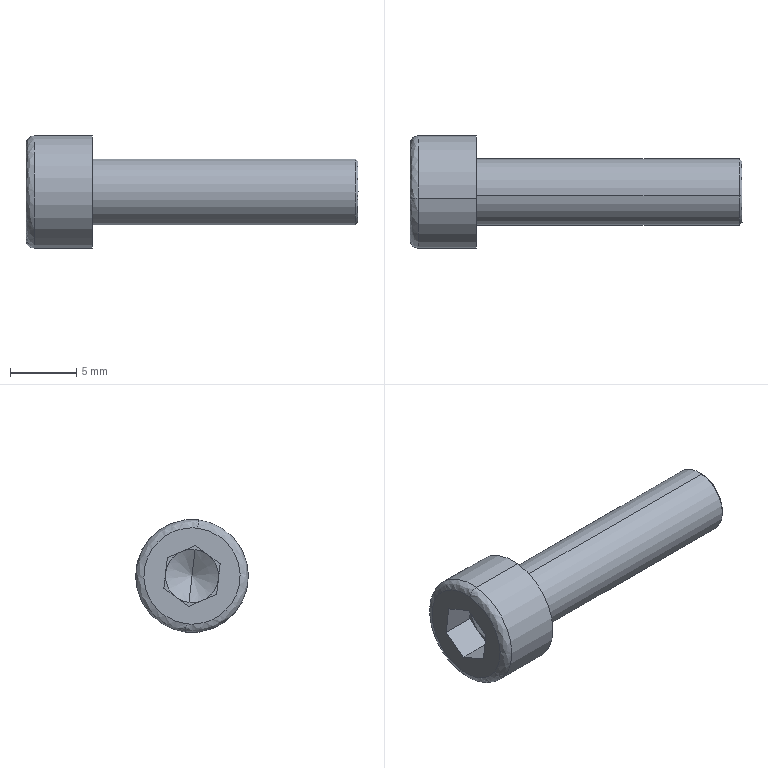Component | SolidWorks | V1ZHXTRR60SecondarySB1-1_v1ZHXTHexagon socket head cap screws GB_GB_FASTENER_SCREWS_HSHCS M5X20-N_1SB1-1 | 1 solid | 25 faces | box 25 x 8.5 x 8.5 mm | volume 634 mm3 | plane 15 | cylinder 4 | cone 4 | spline 2 | commonest cylinder face diameters 5 x2 8.5 x2
STEP:
#1=CARTESIAN_POINT('',(3.529,-7.033,21.044));
#2=VERTEX_POINT('',#1);
#3=CARTESIAN_POINT('',(3.529,-7.072,21.376));
#4=VERTEX_POINT('',#3);
#5=CARTESIAN_POINT('',(3.529,-7.052,21.21));
#6=DIRECTION('',(1.,0.,-0.));
#7=DIRECTION('',(-0.,0.1167,-0.9932));
#8=AXIS2_PLACEMENT_3D('',#5,#6,#7);
#9=CIRCLE('',#8,0.1673);
#10=EDGE_CURVE('',#2,#4,#9,.T.);
#11=ORIENTED_EDGE('',*,*,#10,.F.);
#12=CARTESIAN_POINT('',(3.505,-7.036,21.068));
#13=VERTEX_POINT('',#12);
#14=CARTESIAN_POINT('',(3.529,-7.036,21.068));
#15=DIRECTION('',(-0.,0.9932,0.1167));
#16=DIRECTION('',(-0.,0.1167,-0.9932));
#17=AXIS2_PLACEMENT_3D('',#14,#15,#16);
#18=CIRCLE('',#17,0.02461);
#19=EDGE_CURVE('',#2,#13,#18,.T.);
#20=ORIENTED_EDGE('',*,*,#19,.T.);
#21=CARTESIAN_POINT('',(3.505,-7.069,21.352));
#22=VERTEX_POINT('',#21);
#23=CARTESIAN_POINT('',(3.505,-7.036,21.068));
#24=CARTESIAN_POINT('',(3.505,-6.752,21.102));
#25=CARTESIAN_POINT('',(3.505,-6.786,21.385));
#26=CARTESIAN_POINT('',(3.505,-7.069,21.352));
#27=(BOUNDED_CURVE()B_SPLINE_CURVE(3,(#23,#24,#25,#26),.UNSPECIFIED.,.F.,.F.)B_SPLINE_CURVE_WITH_KNOTS((4,4),(0.,1.),.UNSPECIFIED.)CURVE()GEOMETRIC_REPRESENTATION_ITEM()RATIONAL_B_SPLINE_CURVE((1.,0.3333,0.3333,1.))REPRESENTATION_ITEM(''));
#28=EDGE_CURVE('',#13,#22,#27,.T.);
#29=ORIENTED_EDGE('',*,*,#28,.T.);
#30=CARTESIAN_POINT('',(3.529,-7.069,21.352));
#31=DIRECTION('',(0.,-0.9932,-0.1167));
#32=DIRECTION('',(0.,-0.1167,0.9932));
#33=AXIS2_PLACEMENT_3D('',#30,#31,#32);
#34=CIRCLE('',#33,0.02461);
#35=EDGE_CURVE('',#4,#22,#34,.T.);
#36=ORIENTED_EDGE('',*,*,#35,.F.);
#37=EDGE_LOOP('',(#11,#20,#29,#36));
#38=FACE_OUTER_BOUND('',#37,.T.);
#39=CARTESIAN_POINT('',(3.529,-7.033,21.044));
#40=CARTESIAN_POINT('',(3.529,-6.701,21.083));
#41=CARTESIAN_POINT('',(3.529,-6.74,21.415));
#42=CARTESIAN_POINT('',(3.529,-7.072,21.376));
#43=CARTESIAN_POINT('',(3.515,-7.033,21.044));
#44=CARTESIAN_POINT('',(3.515,-6.701,21.083));
#45=CARTESIAN_POINT('',(3.515,-6.74,21.415));
#46=CARTESIAN_POINT('',(3.515,-7.072,21.376));
#47=CARTESIAN_POINT('',(3.505,-7.034,21.054));
#48=CARTESIAN_POINT('',(3.505,-6.722,21.091));
#49=CARTESIAN_POINT('',(3.505,-6.759,21.403));
#50=CARTESIAN_POINT('',(3.505,-7.071,21.366));
#51=CARTESIAN_POINT('',(3.505,-7.036,21.068));
#52=CARTESIAN_POINT('',(3.505,-6.752,21.102));
#53=CARTESIAN_POINT('',(3.505,-6.786,21.385));
#54=CARTESIAN_POINT('',(3.505,-7.069,21.352));
#55=(BOUNDED_SURFACE()B_SPLINE_SURFACE(3,3,((#39,#40,#41,#42),(#43,#44,#45,#46),(#47,#48,#49,#50),(#51,#52,#53,#54)),.UNSPECIFIED.,.F.,.F.,.F.)B_SPLINE_SURFACE_WITH_KNOTS((4,4),(4,4),(0.,1.),(0.,1.),.UNSPECIFIED.)GEOMETRIC_REPRESENTATION_ITEM()RATIONAL_B_SPLINE_SURFACE(((1.,0.3333,0.3333,1.),(0.8047,0.2682,0.2682,0.8047),(0.8047,0.2682,0.2682,0.8047),(1.,0.3333,0.3333,1.)))REPRESENTATION_ITEM('')SURFACE());
#56=ADVANCED_FACE('',(#38),#55,.T.);
#57=CARTESIAN_POINT('',(4.481,-7.041,21.112));
#58=VERTEX_POINT('',#57);
#59=CARTESIAN_POINT('',(4.481,-7.064,21.308));
#60=VERTEX_POINT('',#59);
#61=CARTESIAN_POINT('',(4.481,-7.052,21.21));
#62=DIRECTION('',(-1.,-0.,0.));
#63=DIRECTION('',(-0.,0.1167,-0.9932));
#64=AXIS2_PLACEMENT_3D('',#61,#62,#63);
#65=CIRCLE('',#64,0.09843);
#66=EDGE_CURVE('',#58,#60,#65,.T.);
#67=ORIENTED_EDGE('',*,*,#66,.T.);
#68=CARTESIAN_POINT('',(3.702,-7.064,21.308));
#69=VERTEX_POINT('',#68);
#70=CARTESIAN_POINT('',(4.489,-7.064,21.308));
#71=DIRECTION('',(-1.,-0.,0.));
#72=VECTOR('',#71,39.37);
#73=LINE('',#70,#72);
#74=EDGE_CURVE('',#60,#69,#73,.T.);
#75=ORIENTED_EDGE('',*,*,#74,.T.);
#76=CARTESIAN_POINT('',(3.702,-7.041,21.112));
#77=VERTEX_POINT('',#76);
#78=CARTESIAN_POINT('',(3.702,-7.052,21.21));
#79=DIRECTION('',(1.,0.,-0.));
#80=DIRECTION('',(-0.,0.1167,-0.9932));
#81=AXIS2_PLACEMENT_3D('',#78,#79,#80);
#82=CIRCLE('',#81,0.09843);
#83=EDGE_CURVE('',#69,#77,#82,.T.);
#84=ORIENTED_EDGE('',*,*,#83,.T.);
#85=CARTESIAN_POINT('',(4.489,-7.041,21.112));
#86=DIRECTION('',(-1.,-0.,0.));
#87=VECTOR('',#86,39.37);
#88=LINE('',#85,#87);
#89=EDGE_CURVE('',#58,#77,#88,.T.);
#90=ORIENTED_EDGE('',*,*,#89,.F.);
#91=EDGE_LOOP('',(#67,#75,#84,#90));
#92=FACE_OUTER_BOUND('',#91,.T.);
#93=CARTESIAN_POINT('',(4.489,-7.052,21.21));
#94=DIRECTION('',(-1.,-0.,0.));
#95=DIRECTION('',(-0.,0.1167,-0.9932));
#96=AXIS2_PLACEMENT_3D('',#93,#94,#95);
#97=CYLINDRICAL_SURFACE('',#96,0.09843);
#98=ADVANCED_FACE('',(#92),#97,.T.);
#99=CARTESIAN_POINT('',(4.489,-7.042,21.12));
#100=VERTEX_POINT('',#99);
#101=CARTESIAN_POINT('',(4.489,-7.063,21.3));
#102=VERTEX_POINT('',#101);
#103=CARTESIAN_POINT('',(4.489,-7.052,21.21));
#104=DIRECTION('',(-1.,-0.,0.));
#105=DIRECTION('',(-0.,0.1167,-0.9932));
#106=AXIS2_PLACEMENT_3D('',#103,#104,#105);
#107=CIRCLE('',#106,0.09055);
#108=EDGE_CURVE('',#100,#102,#107,.T.);
#109=ORIENTED_EDGE('',*,*,#108,.T.);
#110=CARTESIAN_POINT('',(4.481,-7.064,21.308));
#111=DIRECTION('',(-0.7071,-0.0825,0.7023));
#112=VECTOR('',#111,39.37);
#113=LINE('',#110,#112);
#114=EDGE_CURVE('',#102,#60,#113,.T.);
#115=ORIENTED_EDGE('',*,*,#114,.T.);
#116=ORIENTED_EDGE('',*,*,#66,.F.);
#117=CARTESIAN_POINT('',(4.481,-7.041,21.112));
#118=DIRECTION('',(-0.7071,0.0825,-0.7023));
#119=VECTOR('',#118,39.37);
#120=LINE('',#117,#119);
#121=EDGE_CURVE('',#100,#58,#120,.T.);
#122=ORIENTED_EDGE('',*,*,#121,.F.);
#123=EDGE_LOOP('',(#109,#115,#116,#122));
#124=FACE_OUTER_BOUND('',#123,.T.);
#125=CARTESIAN_POINT('',(4.481,-7.052,21.21));
#126=DIRECTION('',(-1.,-0.,0.));
#127=DIRECTION('',(-0.,0.1167,-0.9932));
#128=AXIS2_PLACEMENT_3D('',#125,#126,#127);
#129=CONICAL_SURFACE('',#128,0.09843,0.7854);
#130=ADVANCED_FACE('',(#124),#129,.T.);
#131=CARTESIAN_POINT('',(3.702,-7.072,21.376));
#132=VERTEX_POINT('',#131);
#133=CARTESIAN_POINT('',(3.702,-7.033,21.044));
#134=VERTEX_POINT('',#133);
#135=CARTESIAN_POINT('',(3.702,-7.052,21.21));
#136=DIRECTION('',(1.,0.,-0.));
#137=DIRECTION('',(-0.,0.1167,-0.9932));
#138=AXIS2_PLACEMENT_3D('',#135,#136,#137);
#139=CIRCLE('',#138,0.1673);
#140=EDGE_CURVE('',#132,#134,#139,.T.);
#141=ORIENTED_EDGE('',*,*,#140,.F.);
#142=CARTESIAN_POINT('',(3.702,-7.072,21.376));
#143=DIRECTION('',(-1.,-0.,0.));
#144=VECTOR('',#143,39.37);
#145=LINE('',#142,#144);
#146=EDGE_CURVE('',#132,#4,#145,.T.);
#147=ORIENTED_EDGE('',*,*,#146,.T.);
#148=CARTESIAN_POINT('',(3.529,-7.052,21.21));
#149=DIRECTION('',(1.,0.,-0.));
#150=DIRECTION('',(-0.,0.1167,-0.9932));
#151=AXIS2_PLACEMENT_3D('',#148,#149,#150);
#152=CIRCLE('',#151,0.1673);
#153=EDGE_CURVE('',#4,#2,#152,.T.);
#154=ORIENTED_EDGE('',*,*,#153,.T.);
#155=CARTESIAN_POINT('',(3.702,-7.033,21.044));
#156=DIRECTION('',(-1.,-0.,0.));
#157=VECTOR('',#156,39.37);
#158=LINE('',#155,#157);
#159=EDGE_CURVE('',#134,#2,#158,.T.);
#160=ORIENTED_EDGE('',*,*,#159,.F.);
#161=EDGE_LOOP('',(#141,#147,#154,#160));
#162=FACE_OUTER_BOUND('',#161,.T.);
#163=CARTESIAN_POINT('',(3.702,-7.052,21.21));
#164=DIRECTION('',(-1.,-0.,0.));
#165=DIRECTION('',(-0.,0.1167,-0.9932));
#166=AXIS2_PLACEMENT_3D('',#163,#164,#165);
#167=CYLINDRICAL_SURFACE('',#166,0.1673);
#168=ADVANCED_FACE('',(#162),#167,.T.);
#169=CARTESIAN_POINT('',(3.649,-7.052,21.21));
#170=VERTEX_POINT('',#169);
#171=CARTESIAN_POINT('',(3.603,-7.043,21.132));
#172=VERTEX_POINT('',#171);
#173=CARTESIAN_POINT('',(3.603,-7.043,21.132));
#174=DIRECTION('',(-0.5,0.101,-0.8601));
#175=VECTOR('',#174,39.37);
#176=LINE('',#173,#175);
#177=EDGE_CURVE('',#170,#172,#176,.T.);
#178=ORIENTED_EDGE('',*,*,#177,.F.);
#179=CARTESIAN_POINT('',(3.603,-7.062,21.288));
#180=VERTEX_POINT('',#179);
#181=CARTESIAN_POINT('',(3.603,-7.062,21.288));
#182=DIRECTION('',(-0.5,-0.101,0.8601));
#183=VECTOR('',#182,39.37);
#184=LINE('',#181,#183);
#185=EDGE_CURVE('',#170,#180,#184,.T.);
#186=ORIENTED_EDGE('',*,*,#185,.T.);
#187=CARTESIAN_POINT('',(3.603,-7.021,21.283));
#188=VERTEX_POINT('',#187);
#189=CARTESIAN_POINT('',(3.603,-7.052,21.21));
#190=DIRECTION('',(1.,0.,-0.));
#191=DIRECTION('',(-0.,0.1167,-0.9932));
#192=AXIS2_PLACEMENT_3D('',#189,#190,#191);
#193=CIRCLE('',#192,0.07874);
#194=EDGE_CURVE('',#188,#180,#193,.T.);
#195=ORIENTED_EDGE('',*,*,#194,.F.);
#196=CARTESIAN_POINT('',(3.603,-6.974,21.219));
#197=VERTEX_POINT('',#196);
#198=CARTESIAN_POINT('',(3.603,-7.052,21.21));
#199=DIRECTION('',(1.,0.,-0.));
#200=DIRECTION('',(-0.,0.1167,-0.9932));
#201=AXIS2_PLACEMENT_3D('',#198,#199,#200);
#202=CIRCLE('',#201,0.07874);
#203=EDGE_CURVE('',#197,#188,#202,.T.);
#204=ORIENTED_EDGE('',*,*,#203,.F.);
#205=CARTESIAN_POINT('',(3.603,-7.005,21.147));
#206=VERTEX_POINT('',#205);
#207=CARTESIAN_POINT('',(3.603,-7.052,21.21));
#208=DIRECTION('',(-1.,-0.,0.));
#209=DIRECTION('',(-0.,0.1167,-0.9932));
#210=AXIS2_PLACEMENT_3D('',#207,#208,#209);
#211=CIRCLE('',#210,0.07874);
#212=EDGE_CURVE('',#197,#206,#211,.T.);
#213=ORIENTED_EDGE('',*,*,#212,.T.);
#214=CARTESIAN_POINT('',(3.603,-7.052,21.21));
#215=DIRECTION('',(1.,0.,-0.));
#216=DIRECTION('',(-0.,0.1167,-0.9932));
#217=AXIS2_PLACEMENT_3D('',#214,#215,#216);
#218=CIRCLE('',#217,0.07874);
#219=EDGE_CURVE('',#172,#206,#218,.T.);
#220=ORIENTED_EDGE('',*,*,#219,.F.);
#221=EDGE_LOOP('',(#178,#186,#195,#204,#213,#220));
#222=FACE_OUTER_BOUND('',#221,.T.);
#223=CARTESIAN_POINT('',(3.603,-7.052,21.21));
#224=DIRECTION('',(-1.,-0.,0.));
#225=DIRECTION('',(-0.,0.1167,-0.9932));
#226=AXIS2_PLACEMENT_3D('',#223,#224,#225);
#227=CONICAL_SURFACE('',#226,0.07874,1.047);
#228=ADVANCED_FACE('',(#222),#227,.F.);
#229=ORIENTED_EDGE('',*,*,#74,.F.);
#230=CARTESIAN_POINT('',(4.481,-7.052,21.21));
#231=DIRECTION('',(-1.,-0.,0.));
#232=DIRECTION('',(-0.,0.1167,-0.9932));
#233=AXIS2_PLACEMENT_3D('',#230,#231,#232);
#234=CIRCLE('',#233,0.09843);
#235=EDGE_CURVE('',#60,#58,#234,.T.);
#236=ORIENTED_EDGE('',*,*,#235,.T.);
#237=ORIENTED_EDGE('',*,*,#89,.T.);
#238=CARTESIAN_POINT('',(3.702,-7.052,21.21));
#239=DIRECTION('',(1.,0.,-0.));
#240=DIRECTION('',(-0.,0.1167,-0.9932));
#241=AXIS2_PLACEMENT_3D('',#238,#239,#240);
#242=CIRCLE('',#241,0.09843);
#243=EDGE_CURVE('',#77,#69,#242,.T.);
#244=ORIENTED_EDGE('',*,*,#243,.T.);
#245=EDGE_LOOP('',(#229,#236,#237,#244));
#246=FACE_OUTER_BOUND('',#245,.T.);
#247=CARTESIAN_POINT('',(4.489,-7.052,21.21));
#248=DIRECTION('',(-1.,-0.,0.));
#249=DIRECTION('',(-0.,0.1167,-0.9932));
#250=AXIS2_PLACEMENT_3D('',#247,#248,#249);
#251=CYLINDRICAL_SURFACE('',#250,0.09843);
#252=ADVANCED_FACE('',(#246),#251,.T.);
#253=ORIENTED_EDGE('',*,*,#243,.F.);
#254=ORIENTED_EDGE('',*,*,#83,.F.);
#255=EDGE_LOOP('',(#253,#254));
#256=FACE_BOUND('',#255,.T.);
#257=CARTESIAN_POINT('',(3.702,-7.052,21.21));
#258=DIRECTION('',(1.,0.,-0.));
#259=DIRECTION('',(-0.,0.1167,-0.9932));
#260=AXIS2_PLACEMENT_3D('',#257,#258,#259);
#261=CIRCLE('',#260,0.1673);
#262=EDGE_CURVE('',#134,#132,#261,.T.);
#263=ORIENTED_EDGE('',*,*,#262,.T.);
#264=ORIENTED_EDGE('',*,*,#140,.T.);
#265=EDGE_LOOP('',(#263,#264));
#266=FACE_OUTER_BOUND('',#265,.T.);
#267=CARTESIAN_POINT('',(3.702,-7.052,21.21));
#268=DIRECTION('',(1.,0.,-0.));
#269=DIRECTION('',(0.,-0.1167,0.9932));
#270=AXIS2_PLACEMENT_3D('',#267,#268,#269);
#271=PLANE('',#270);
#272=ADVANCED_FACE('',(#256,#266),#271,.T.);
#273=ORIENTED_EDGE('',*,*,#114,.F.);
#274=CARTESIAN_POINT('',(4.489,-7.052,21.21));
#275=DIRECTION('',(-1.,-0.,0.));
#276=DIRECTION('',(-0.,0.1167,-0.9932));
#277=AXIS2_PLACEMENT_3D('',#274,#275,#276);
#278=CIRCLE('',#277,0.09055);
#279=EDGE_CURVE('',#102,#100,#278,.T.);
#280=ORIENTED_EDGE('',*,*,#279,.T.);
#281=ORIENTED_EDGE('',*,*,#121,.T.);
#282=ORIENTED_EDGE('',*,*,#235,.F.);
#283=EDGE_LOOP('',(#273,#280,#281,#282));
#284=FACE_OUTER_BOUND('',#283,.T.);
#285=CARTESIAN_POINT('',(4.481,-7.052,21.21));
#286=DIRECTION('',(-1.,-0.,0.));
#287=DIRECTION('',(-0.,0.1167,-0.9932));
#288=AXIS2_PLACEMENT_3D('',#285,#286,#287);
#289=CONICAL_SURFACE('',#288,0.09843,0.7854);
#290=ADVANCED_FACE('',(#284),#289,.T.);
#291=ORIENTED_EDGE('',*,*,#146,.F.);
#292=ORIENTED_EDGE('',*,*,#262,.F.);
#293=ORIENTED_EDGE('',*,*,#159,.T.);
#294=ORIENTED_EDGE('',*,*,#10,.T.);
#295=EDGE_LOOP('',(#291,#292,#293,#294));
#296=FACE_OUTER_BOUND('',#295,.T.);
#297=CARTESIAN_POINT('',(3.702,-7.052,21.21));
#298=DIRECTION('',(-1.,-0.,0.));
#299=DIRECTION('',(-0.,0.1167,-0.9932));
#300=AXIS2_PLACEMENT_3D('',#297,#298,#299);
#301=CYLINDRICAL_SURFACE('',#300,0.1673);
#302=ADVANCED_FACE('',(#296),#301,.T.);
#303=ORIENTED_EDGE('',*,*,#108,.F.);
#304=ORIENTED_EDGE('',*,*,#279,.F.);
#305=EDGE_LOOP('',(#303,#304));
#306=FACE_OUTER_BOUND('',#305,.T.);
#307=CARTESIAN_POINT('',(4.489,-7.052,21.21));
#308=DIRECTION('',(1.,0.,-0.));
#309=DIRECTION('',(0.,-0.1167,0.9932));
#310=AXIS2_PLACEMENT_3D('',#307,#308,#309);
#311=PLANE('',#310);
#312=ADVANCED_FACE('',(#306),#311,.T.);
#313=ORIENTED_EDGE('',*,*,#19,.F.);
#314=ORIENTED_EDGE('',*,*,#153,.F.);
#315=ORIENTED_EDGE('',*,*,#35,.T.);
#316=CARTESIAN_POINT('',(3.505,-7.069,21.352));
#317=CARTESIAN_POINT('',(3.505,-7.353,21.319));
#318=CARTESIAN_POINT('',(3.505,-7.319,21.035));
#319=CARTESIAN_POINT('',(3.505,-7.036,21.068));
#320=(BOUNDED_CURVE()B_SPLINE_CURVE(3,(#316,#317,#318,#319),.UNSPECIFIED.,.F.,.F.)B_SPLINE_CURVE_WITH_KNOTS((4,4),(0.,1.),.UNSPECIFIED.)CURVE()GEOMETRIC_REPRESENTATION_ITEM()RATIONAL_B_SPLINE_CURVE((1.,0.3333,0.3333,1.))REPRESENTATION_ITEM(''));
#321=EDGE_CURVE('',#22,#13,#320,.T.);
#322=ORIENTED_EDGE('',*,*,#321,.T.);
#323=EDGE_LOOP('',(#313,#314,#315,#322));
#324=FACE_OUTER_BOUND('',#323,.T.);
#325=CARTESIAN_POINT('',(3.529,-7.072,21.376));
#326=CARTESIAN_POINT('',(3.529,-7.404,21.337));
#327=CARTESIAN_POINT('',(3.529,-7.365,21.005));
#328=CARTESIAN_POINT('',(3.529,-7.033,21.044));
#329=CARTESIAN_POINT('',(3.515,-7.072,21.376));
#330=CARTESIAN_POINT('',(3.515,-7.404,21.337));
#331=CARTESIAN_POINT('',(3.515,-7.365,21.005));
#332=CARTESIAN_POINT('',(3.515,-7.033,21.044));
#333=CARTESIAN_POINT('',(3.505,-7.071,21.366));
#334=CARTESIAN_POINT('',(3.505,-7.383,21.33));
#335=CARTESIAN_POINT('',(3.505,-7.346,21.017));
#336=CARTESIAN_POINT('',(3.505,-7.034,21.054));
#337=CARTESIAN_POINT('',(3.505,-7.069,21.352));
#338=CARTESIAN_POINT('',(3.505,-7.353,21.319));
#339=CARTESIAN_POINT('',(3.505,-7.319,21.035));
#340=CARTESIAN_POINT('',(3.505,-7.036,21.068));
#341=(BOUNDED_SURFACE()B_SPLINE_SURFACE(3,3,((#325,#326,#327,#328),(#329,#330,#331,#332),(#333,#334,#335,#336),(#337,#338,#339,#340)),.UNSPECIFIED.,.F.,.F.,.T.)B_SPLINE_SURFACE_WITH_KNOTS((4,4),(4,4),(0.,1.),(0.,1.),.UNSPECIFIED.)GEOMETRIC_REPRESENTATION_ITEM()RATIONAL_B_SPLINE_SURFACE(((1.,0.3333,0.3333,1.),(0.8047,0.2682,0.2682,0.8047),(0.8047,0.2682,0.2682,0.8047),(1.,0.3333,0.3333,1.)))REPRESENTATION_ITEM('')SURFACE());
#342=ADVANCED_FACE('',(#324),#341,.T.);
#343=CARTESIAN_POINT('',(3.505,-7.136,21.246));
#344=VERTEX_POINT('',#343);
#345=CARTESIAN_POINT('',(3.505,-7.063,21.301));
#346=VERTEX_POINT('',#345);
#347=CARTESIAN_POINT('',(3.505,-7.136,21.246));
#348=DIRECTION('',(-0.,0.8018,0.5976));
#349=VECTOR('',#348,39.37);
#350=LINE('',#347,#349);
#351=EDGE_CURVE('',#344,#346,#350,.T.);
#352=ORIENTED_EDGE('',*,*,#351,.F.);
#353=CARTESIAN_POINT('',(3.505,-7.125,21.156));
#354=VERTEX_POINT('',#353);
#355=CARTESIAN_POINT('',(3.505,-7.131,21.201));
#356=DIRECTION('',(0.,-0.1167,0.9932));
#357=VECTOR('',#356,39.37);
#358=LINE('',#355,#357);
#359=EDGE_CURVE('',#354,#344,#358,.T.);
#360=ORIENTED_EDGE('',*,*,#359,.F.);
#361=CARTESIAN_POINT('',(3.505,-7.042,21.12));
#362=VERTEX_POINT('',#361);
#363=CARTESIAN_POINT('',(3.505,-7.042,21.12));
#364=DIRECTION('',(0.,-0.9184,0.3955));
#365=VECTOR('',#364,39.37);
#366=LINE('',#363,#365);
#367=EDGE_CURVE('',#362,#354,#366,.T.);
#368=ORIENTED_EDGE('',*,*,#367,.F.);
#369=CARTESIAN_POINT('',(3.505,-6.969,21.174));
#370=VERTEX_POINT('',#369);
#371=CARTESIAN_POINT('',(3.505,-6.969,21.174));
#372=DIRECTION('',(0.,-0.8018,-0.5976));
#373=VECTOR('',#372,39.37);
#374=LINE('',#371,#373);
#375=EDGE_CURVE('',#370,#362,#374,.T.);
#376=ORIENTED_EDGE('',*,*,#375,.F.);
#377=CARTESIAN_POINT('',(3.505,-6.98,21.265));
#378=VERTEX_POINT('',#377);
#379=CARTESIAN_POINT('',(3.505,-6.974,21.219));
#380=DIRECTION('',(-0.,0.1167,-0.9932));
#381=VECTOR('',#380,39.37);
#382=LINE('',#379,#381);
#383=EDGE_CURVE('',#378,#370,#382,.T.);
#384=ORIENTED_EDGE('',*,*,#383,.F.);
#385=CARTESIAN_POINT('',(3.505,-7.063,21.301));
#386=DIRECTION('',(-0.,0.9184,-0.3955));
#387=VECTOR('',#386,39.37);
#388=LINE('',#385,#387);
#389=EDGE_CURVE('',#346,#378,#388,.T.);
#390=ORIENTED_EDGE('',*,*,#389,.F.);
#391=EDGE_LOOP('',(#352,#360,#368,#376,#384,#390));
#392=FACE_BOUND('',#391,.T.);
#393=ORIENTED_EDGE('',*,*,#321,.F.);
#394=ORIENTED_EDGE('',*,*,#28,.F.);
#395=EDGE_LOOP('',(#393,#394));
#396=FACE_OUTER_BOUND('',#395,.T.);
#397=CARTESIAN_POINT('',(3.505,-7.052,21.21));
#398=DIRECTION('',(1.,0.,-0.));
#399=DIRECTION('',(0.,-0.1167,0.9932));
#400=AXIS2_PLACEMENT_3D('',#397,#398,#399);
#401=PLANE('',#400);
#402=ADVANCED_FACE('',(#392,#396),#401,.F.);
#403=CARTESIAN_POINT('',(3.603,-7.063,21.301));
#404=VERTEX_POINT('',#403);
#405=CARTESIAN_POINT('',(3.603,-6.98,21.265));
#406=DIRECTION('',(0.,-0.9184,0.3955));
#407=VECTOR('',#406,39.37);
#408=LINE('',#405,#407);
#409=EDGE_CURVE('',#188,#404,#408,.T.);
#410=ORIENTED_EDGE('',*,*,#409,.T.);
#411=CARTESIAN_POINT('',(3.603,-7.063,21.301));
#412=DIRECTION('',(-1.,-0.,0.));
#413=VECTOR('',#412,39.37);
#414=LINE('',#411,#413);
#415=EDGE_CURVE('',#404,#346,#414,.T.);
#416=ORIENTED_EDGE('',*,*,#415,.T.);
#417=ORIENTED_EDGE('',*,*,#389,.T.);
#418=CARTESIAN_POINT('',(3.603,-6.98,21.265));
#419=VERTEX_POINT('',#418);
#420=CARTESIAN_POINT('',(3.603,-6.98,21.265));
#421=DIRECTION('',(1.,0.,-0.));
#422=VECTOR('',#421,39.37);
#423=LINE('',#420,#422);
#424=EDGE_CURVE('',#378,#419,#423,.T.);
#425=ORIENTED_EDGE('',*,*,#424,.T.);
#426=CARTESIAN_POINT('',(3.603,-6.98,21.265));
#427=DIRECTION('',(0.,-0.9184,0.3955));
#428=VECTOR('',#427,39.37);
#429=LINE('',#426,#428);
#430=EDGE_CURVE('',#419,#188,#429,.T.);
#431=ORIENTED_EDGE('',*,*,#430,.T.);
#432=EDGE_LOOP('',(#410,#416,#417,#425,#431));
#433=FACE_OUTER_BOUND('',#432,.T.);
#434=CARTESIAN_POINT('',(3.603,-6.98,21.265));
#435=DIRECTION('',(0.,-0.3955,-0.9184));
#436=DIRECTION('',(-0.,0.9184,-0.3955));
#437=AXIS2_PLACEMENT_3D('',#434,#435,#436);
#438=PLANE('',#437);
#439=ADVANCED_FACE('',(#433),#438,.T.);
#440=CARTESIAN_POINT('',(3.603,-7.099,21.273));
#441=VERTEX_POINT('',#440);
#442=CARTESIAN_POINT('',(3.603,-7.136,21.246));
#443=VERTEX_POINT('',#442);
#444=CARTESIAN_POINT('',(3.603,-7.099,21.273));
#445=DIRECTION('',(0.,-0.8018,-0.5976));
#446=VECTOR('',#445,39.37);
#447=LINE('',#444,#446);
#448=EDGE_CURVE('',#441,#443,#447,.T.);
#449=ORIENTED_EDGE('',*,*,#448,.T.);
#450=CARTESIAN_POINT('',(3.603,-7.136,21.246));
#451=DIRECTION('',(-1.,-0.,0.));
#452=VECTOR('',#451,39.37);
#453=LINE('',#450,#452);
#454=EDGE_CURVE('',#443,#344,#453,.T.);
#455=ORIENTED_EDGE('',*,*,#454,.T.);
#456=ORIENTED_EDGE('',*,*,#351,.T.);
#457=ORIENTED_EDGE('',*,*,#415,.F.);
#458=CARTESIAN_POINT('',(3.603,-7.063,21.301));
#459=DIRECTION('',(0.,-0.8018,-0.5976));
#460=VECTOR('',#459,39.37);
#461=LINE('',#458,#460);
#462=EDGE_CURVE('',#404,#441,#461,.T.);
#463=ORIENTED_EDGE('',*,*,#462,.T.);
#464=EDGE_LOOP('',(#449,#455,#456,#457,#463));
#465=FACE_OUTER_BOUND('',#464,.T.);
#466=CARTESIAN_POINT('',(3.603,-7.063,21.301));
#467=DIRECTION('',(-0.,0.5976,-0.8018));
#468=DIRECTION('',(-0.,0.8018,0.5976));
#469=AXIS2_PLACEMENT_3D('',#466,#467,#468);
#470=PLANE('',#469);
#471=ADVANCED_FACE('',(#465),#470,.T.);
#472=CARTESIAN_POINT('',(3.603,-7.131,21.201));
#473=VERTEX_POINT('',#472);
#474=CARTESIAN_POINT('',(3.603,-7.125,21.156));
#475=VERTEX_POINT('',#474);
#476=CARTESIAN_POINT('',(3.603,-7.141,21.291));
#477=DIRECTION('',(-0.,0.1167,-0.9932));
#478=VECTOR('',#477,39.37);
#479=LINE('',#476,#478);
#480=EDGE_CURVE('',#473,#475,#479,.T.);
#481=ORIENTED_EDGE('',*,*,#480,.T.);
#482=CARTESIAN_POINT('',(3.603,-7.125,21.156));
#483=DIRECTION('',(-1.,-0.,0.));
#484=VECTOR('',#483,39.37);
#485=LINE('',#482,#484);
#486=EDGE_CURVE('',#475,#354,#485,.T.);
#487=ORIENTED_EDGE('',*,*,#486,.T.);
#488=ORIENTED_EDGE('',*,*,#359,.T.);
#489=ORIENTED_EDGE('',*,*,#454,.F.);
#490=CARTESIAN_POINT('',(3.603,-7.141,21.291));
#491=DIRECTION('',(-0.,0.1167,-0.9932));
#492=VECTOR('',#491,39.37);
#493=LINE('',#490,#492);
#494=EDGE_CURVE('',#443,#473,#493,.T.);
#495=ORIENTED_EDGE('',*,*,#494,.T.);
#496=EDGE_LOOP('',(#481,#487,#488,#489,#495));
#497=FACE_OUTER_BOUND('',#496,.T.);
#498=CARTESIAN_POINT('',(3.603,-7.136,21.246));
#499=DIRECTION('',(-0.,0.9932,0.1167));
#500=DIRECTION('',(0.,-0.1167,0.9932));
#501=AXIS2_PLACEMENT_3D('',#498,#499,#500);
#502=PLANE('',#501);
#503=ADVANCED_FACE('',(#497),#502,.T.);
#504=CARTESIAN_POINT('',(3.603,-7.084,21.138));
#505=VERTEX_POINT('',#504);
#506=CARTESIAN_POINT('',(3.603,-7.042,21.12));
#507=VERTEX_POINT('',#506);
#508=CARTESIAN_POINT('',(3.603,-7.125,21.156));
#509=DIRECTION('',(-0.,0.9184,-0.3955));
#510=VECTOR('',#509,39.37);
#511=LINE('',#508,#510);
#512=EDGE_CURVE('',#505,#507,#511,.T.);
#513=ORIENTED_EDGE('',*,*,#512,.T.);
#514=CARTESIAN_POINT('',(3.603,-7.042,21.12));
#515=DIRECTION('',(-1.,-0.,0.));
#516=VECTOR('',#515,39.37);
#517=LINE('',#514,#516);
#518=EDGE_CURVE('',#507,#362,#517,.T.);
#519=ORIENTED_EDGE('',*,*,#518,.T.);
#520=ORIENTED_EDGE('',*,*,#367,.T.);
#521=ORIENTED_EDGE('',*,*,#486,.F.);
#522=CARTESIAN_POINT('',(3.603,-7.125,21.156));
#523=DIRECTION('',(-0.,0.9184,-0.3955));
#524=VECTOR('',#523,39.37);
#525=LINE('',#522,#524);
#526=EDGE_CURVE('',#475,#505,#525,.T.);
#527=ORIENTED_EDGE('',*,*,#526,.T.);
#528=EDGE_LOOP('',(#513,#519,#520,#521,#527));
#529=FACE_OUTER_BOUND('',#528,.T.);
#530=CARTESIAN_POINT('',(3.603,-7.125,21.156));
#531=DIRECTION('',(-0.,0.3955,0.9184));
#532=DIRECTION('',(0.,-0.9184,0.3955));
#533=AXIS2_PLACEMENT_3D('',#530,#531,#532);
#534=PLANE('',#533);
#535=ADVANCED_FACE('',(#529),#534,.T.);
#536=CARTESIAN_POINT('',(3.603,-6.969,21.174));
#537=VERTEX_POINT('',#536);
#538=CARTESIAN_POINT('',(3.603,-7.042,21.12));
#539=DIRECTION('',(-0.,0.8018,0.5976));
#540=VECTOR('',#539,39.37);
#541=LINE('',#538,#540);
#542=EDGE_CURVE('',#206,#537,#541,.T.);
#543=ORIENTED_EDGE('',*,*,#542,.T.);
#544=CARTESIAN_POINT('',(3.603,-6.969,21.174));
#545=DIRECTION('',(-1.,-0.,0.));
#546=VECTOR('',#545,39.37);
#547=LINE('',#544,#546);
#548=EDGE_CURVE('',#537,#370,#547,.T.);
#549=ORIENTED_EDGE('',*,*,#548,.T.);
#550=ORIENTED_EDGE('',*,*,#375,.T.);
#551=ORIENTED_EDGE('',*,*,#518,.F.);
#552=CARTESIAN_POINT('',(3.603,-7.042,21.12));
#553=DIRECTION('',(-0.,0.8018,0.5976));
#554=VECTOR('',#553,39.37);
#555=LINE('',#552,#554);
#556=EDGE_CURVE('',#507,#206,#555,.T.);
#557=ORIENTED_EDGE('',*,*,#556,.T.);
#558=EDGE_LOOP('',(#543,#549,#550,#551,#557));
#559=FACE_OUTER_BOUND('',#558,.T.);
#560=CARTESIAN_POINT('',(3.603,-7.042,21.12));
#561=DIRECTION('',(0.,-0.5976,0.8018));
#562=DIRECTION('',(0.,-0.8018,-0.5976));
#563=AXIS2_PLACEMENT_3D('',#560,#561,#562);
#564=PLANE('',#563);
#565=ADVANCED_FACE('',(#559),#564,.T.);
#566=CARTESIAN_POINT('',(3.603,-6.985,21.31));
#567=DIRECTION('',(0.,-0.1167,0.9932));
#568=VECTOR('',#567,39.37);
#569=LINE('',#566,#568);
#570=EDGE_CURVE('',#197,#419,#569,.T.);
#571=ORIENTED_EDGE('',*,*,#570,.T.);
#572=ORIENTED_EDGE('',*,*,#424,.F.);
#573=ORIENTED_EDGE('',*,*,#383,.T.);
#574=ORIENTED_EDGE('',*,*,#548,.F.);
#575=CARTESIAN_POINT('',(3.603,-6.969,21.174));
#576=DIRECTION('',(0.,-0.1167,0.9932));
#577=VECTOR('',#576,39.37);
#578=LINE('',#575,#577);
#579=EDGE_CURVE('',#537,#197,#578,.T.);
#580=ORIENTED_EDGE('',*,*,#579,.T.);
#581=EDGE_LOOP('',(#571,#572,#573,#574,#580));
#582=FACE_OUTER_BOUND('',#581,.T.);
#583=CARTESIAN_POINT('',(3.603,-6.969,21.174));
#584=DIRECTION('',(0.,-0.9932,-0.1167));
#585=DIRECTION('',(-0.,0.1167,-0.9932));
#586=AXIS2_PLACEMENT_3D('',#583,#584,#585);
#587=PLANE('',#586);
#588=ADVANCED_FACE('',(#582),#587,.T.);
#589=ORIENTED_EDGE('',*,*,#462,.F.);
#590=ORIENTED_EDGE('',*,*,#409,.F.);
#591=ORIENTED_EDGE('',*,*,#194,.T.);
#592=CARTESIAN_POINT('',(3.603,-7.052,21.21));
#593=DIRECTION('',(1.,0.,-0.));
#594=DIRECTION('',(-0.,0.1167,-0.9932));
#595=AXIS2_PLACEMENT_3D('',#592,#593,#594);
#596=CIRCLE('',#595,0.07874);
#597=EDGE_CURVE('',#180,#441,#596,.T.);
#598=ORIENTED_EDGE('',*,*,#597,.T.);
#599=EDGE_LOOP('',(#589,#590,#591,#598));
#600=FACE_OUTER_BOUND('',#599,.T.);
#601=CARTESIAN_POINT('',(3.603,-7.063,21.301));
#602=DIRECTION('',(1.,0.,-0.));
#603=DIRECTION('',(0.,-0.1167,0.9932));
#604=AXIS2_PLACEMENT_3D('',#601,#602,#603);
#605=PLANE('',#604);
#606=ADVANCED_FACE('',(#600),#605,.F.);
#607=ORIENTED_EDGE('',*,*,#556,.F.);
#608=ORIENTED_EDGE('',*,*,#512,.F.);
#609=CARTESIAN_POINT('',(3.603,-7.052,21.21));
#610=DIRECTION('',(1.,0.,-0.));
#611=DIRECTION('',(-0.,0.1167,-0.9932));
#612=AXIS2_PLACEMENT_3D('',#609,#610,#611);
#613=CIRCLE('',#612,0.07874);
#614=EDGE_CURVE('',#505,#172,#613,.T.);
#615=ORIENTED_EDGE('',*,*,#614,.T.);
#616=ORIENTED_EDGE('',*,*,#219,.T.);
#617=EDGE_LOOP('',(#607,#608,#615,#616));
#618=FACE_OUTER_BOUND('',#617,.T.);
#619=CARTESIAN_POINT('',(3.603,-7.063,21.301));
#620=DIRECTION('',(1.,0.,-0.));
#621=DIRECTION('',(0.,-0.1167,0.9932));
#622=AXIS2_PLACEMENT_3D('',#619,#620,#621);
#623=PLANE('',#622);
#624=ADVANCED_FACE('',(#618),#623,.F.);
#625=ORIENTED_EDGE('',*,*,#579,.F.);
#626=ORIENTED_EDGE('',*,*,#542,.F.);
#627=ORIENTED_EDGE('',*,*,#212,.F.);
#628=EDGE_LOOP('',(#625,#626,#627));
#629=FACE_OUTER_BOUND('',#628,.T.);
#630=CARTESIAN_POINT('',(3.603,-7.063,21.301));
#631=DIRECTION('',(1.,0.,-0.));
#632=DIRECTION('',(0.,-0.1167,0.9932));
#633=AXIS2_PLACEMENT_3D('',#630,#631,#632);
#634=PLANE('',#633);
#635=ADVANCED_FACE('',(#629),#634,.F.);
#636=ORIENTED_EDGE('',*,*,#185,.F.);
#637=ORIENTED_EDGE('',*,*,#177,.T.);
#638=ORIENTED_EDGE('',*,*,#614,.F.);
#639=CARTESIAN_POINT('',(3.603,-7.052,21.21));
#640=DIRECTION('',(1.,0.,-0.));
#641=DIRECTION('',(-0.,0.1167,-0.9932));
#642=AXIS2_PLACEMENT_3D('',#639,#640,#641);
#643=CIRCLE('',#642,0.07874);
#644=EDGE_CURVE('',#473,#505,#643,.T.);
#645=ORIENTED_EDGE('',*,*,#644,.F.);
#646=CARTESIAN_POINT('',(3.603,-7.052,21.21));
#647=DIRECTION('',(1.,0.,-0.));
#648=DIRECTION('',(-0.,0.1167,-0.9932));
#649=AXIS2_PLACEMENT_3D('',#646,#647,#648);
#650=CIRCLE('',#649,0.07874);
#651=EDGE_CURVE('',#441,#473,#650,.T.);
#652=ORIENTED_EDGE('',*,*,#651,.F.);
#653=ORIENTED_EDGE('',*,*,#597,.F.);
#654=EDGE_LOOP('',(#636,#637,#638,#645,#652,#653));
#655=FACE_OUTER_BOUND('',#654,.T.);
#656=CARTESIAN_POINT('',(3.603,-7.052,21.21));
#657=DIRECTION('',(-1.,-0.,0.));
#658=DIRECTION('',(-0.,0.1167,-0.9932));
#659=AXIS2_PLACEMENT_3D('',#656,#657,#658);
#660=CONICAL_SURFACE('',#659,0.07874,1.047);
#661=ADVANCED_FACE('',(#655),#660,.F.);
#662=ORIENTED_EDGE('',*,*,#430,.F.);
#663=ORIENTED_EDGE('',*,*,#570,.F.);
#664=ORIENTED_EDGE('',*,*,#203,.T.);
#665=EDGE_LOOP('',(#662,#663,#664));
#666=FACE_OUTER_BOUND('',#665,.T.);
#667=CARTESIAN_POINT('',(3.603,-7.063,21.301));
#668=DIRECTION('',(1.,0.,-0.));
#669=DIRECTION('',(0.,-0.1167,0.9932));
#670=AXIS2_PLACEMENT_3D('',#667,#668,#669);
#671=PLANE('',#670);
#672=ADVANCED_FACE('',(#666),#671,.F.);
#673=ORIENTED_EDGE('',*,*,#526,.F.);
#674=ORIENTED_EDGE('',*,*,#480,.F.);
#675=ORIENTED_EDGE('',*,*,#644,.T.);
#676=EDGE_LOOP('',(#673,#674,#675));
#677=FACE_OUTER_BOUND('',#676,.T.);
#678=CARTESIAN_POINT('',(3.603,-7.063,21.301));
#679=DIRECTION('',(1.,0.,-0.));
#680=DIRECTION('',(0.,-0.1167,0.9932));
#681=AXIS2_PLACEMENT_3D('',#678,#679,#680);
#682=PLANE('',#681);
#683=ADVANCED_FACE('',(#677),#682,.F.);
#684=ORIENTED_EDGE('',*,*,#494,.F.);
#685=ORIENTED_EDGE('',*,*,#448,.F.);
#686=ORIENTED_EDGE('',*,*,#651,.T.);
#687=EDGE_LOOP('',(#684,#685,#686));
#688=FACE_OUTER_BOUND('',#687,.T.);
#689=CARTESIAN_POINT('',(3.603,-7.063,21.301));
#690=DIRECTION('',(1.,0.,-0.));
#691=DIRECTION('',(0.,-0.1167,0.9932));
#692=AXIS2_PLACEMENT_3D('',#689,#690,#691);
#693=PLANE('',#692);
#694=ADVANCED_FACE('',(#688),#693,.F.);
#695=CLOSED_SHELL('',(#56,#98,#130,#168,#228,#252,#272,#290,#302,#312,#342,#402,#439,#471,#503,#535,#565,#588,#606,#624,#635,#661,#672,#683,#694));
#696=MANIFOLD_SOLID_BREP('',#695);
#697=CARTESIAN_POINT('',(0.,0.,0.));
#698=DIRECTION('',(0.,0.,1.));
#699=DIRECTION('',(1.,0.,0.));
#700=AXIS2_PLACEMENT_3D('',#697,#698,#699);
#701=(LENGTH_UNIT()NAMED_UNIT(*)SI_UNIT($,.METRE.));
#702=LENGTH_MEASURE_WITH_UNIT(LENGTH_MEASURE(0.0254),#701);
#703=DIMENSIONAL_EXPONENTS(1.,0.,0.,0.,0.,0.,0.);
#704=(CONVERSION_BASED_UNIT('',#702)LENGTH_UNIT()NAMED_UNIT(#703));
#705=UNCERTAINTY_MEASURE_WITH_UNIT(LENGTH_MEASURE(0.00001),#704,'','');
#706=(NAMED_UNIT(*)PLANE_ANGLE_UNIT()SI_UNIT($,.RADIAN.));
#707=(NAMED_UNIT(*)SI_UNIT($,.STERADIAN.)SOLID_ANGLE_UNIT());
#708=(GEOMETRIC_REPRESENTATION_CONTEXT(3)GLOBAL_UNCERTAINTY_ASSIGNED_CONTEXT((#705))GLOBAL_UNIT_ASSIGNED_CONTEXT((#704,#706,#707))REPRESENTATION_CONTEXT('',''));
#709=ADVANCED_BREP_SHAPE_REPRESENTATION('',(#696,#700),#708);
#710=COLOUR_RGB('',0.7922,0.8196,0.9333);
#711=FILL_AREA_STYLE_COLOUR('',#710);
#712=FILL_AREA_STYLE('',(#711));
#713=SURFACE_STYLE_FILL_AREA(#712);
#714=SURFACE_SIDE_STYLE('',(#713));
#715=SURFACE_STYLE_USAGE(.BOTH.,#714);
#716=PRESENTATION_STYLE_ASSIGNMENT((#715));
#717=STYLED_ITEM('',(#716),#696);
#718=PRESENTATION_LAYER_ASSIGNMENT('','',(#717));
#719=(LENGTH_UNIT()NAMED_UNIT(*)SI_UNIT($,.METRE.));
#720=LENGTH_MEASURE_WITH_UNIT(LENGTH_MEASURE(0.0254),#719);
#721=DIMENSIONAL_EXPONENTS(1.,0.,0.,0.,0.,0.,0.);
#722=(CONVERSION_BASED_UNIT('',#720)LENGTH_UNIT()NAMED_UNIT(#721));
#723=UNCERTAINTY_MEASURE_WITH_UNIT(LENGTH_MEASURE(0.00001),#722,'','');
#724=(NAMED_UNIT(*)PLANE_ANGLE_UNIT()SI_UNIT($,.RADIAN.));
#725=(NAMED_UNIT(*)SI_UNIT($,.STERADIAN.)SOLID_ANGLE_UNIT());
#726=(GEOMETRIC_REPRESENTATION_CONTEXT(3)GLOBAL_UNCERTAINTY_ASSIGNED_CONTEXT((#723))GLOBAL_UNIT_ASSIGNED_CONTEXT((#722,#724,#725))REPRESENTATION_CONTEXT('',''));
#727=MECHANICAL_DESIGN_GEOMETRIC_PRESENTATION_REPRESENTATION('',(#717),#726);